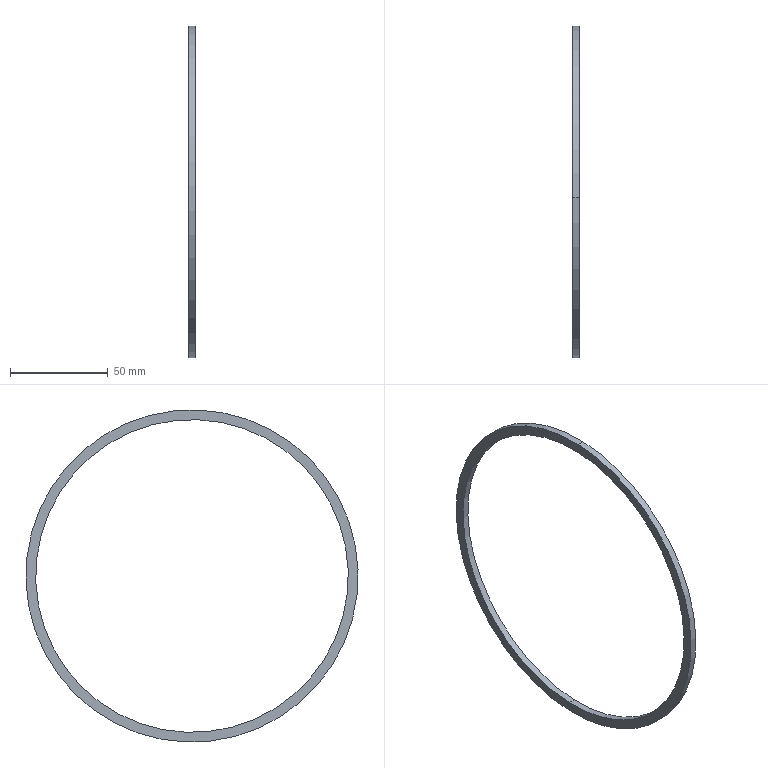Component | SolidWorks | SealRing2-1 | 1 solid | 6 faces | box 3.5 x 170 x 170 mm | volume 9071 mm3 | cylinder 4 | plane 2 | commonest cylinder face diameters 160 x2 170 x2
build123d program:
from build123d import *

# Parameters (mm, degrees)
SKETCH2_R           = 85
SKETCH2_R_2         = 80
BOSS_EXTRUDE1_DEPTH = 3.5


with BuildPart() as part:
    # Sketch2 → Boss-Extrude1 (new body)
    with BuildSketch(Plane(origin=(0, 0, 0), x_dir=(0, 0, -1), z_dir=(1, 0, 0))):
        Circle(SKETCH2_R)
        Circle(SKETCH2_R_2, mode=Mode.SUBTRACT)
    extrude(amount=BOSS_EXTRUDE1_DEPTH)


solid = part.part

# Placed as in the assembly
solid = solid.moved(Location((-63.5, 0, 0), (0, 0, 0)))
STEP:
#1=CARTESIAN_POINT('',(-2.362,-0.1192,3.147));
#2=VERTEX_POINT('',#1);
#3=CARTESIAN_POINT('',(-2.362,0.1192,-3.147));
#4=VERTEX_POINT('',#3);
#5=CARTESIAN_POINT('',(-2.362,-0.,-0.));
#6=DIRECTION('',(1.,0.,0.));
#7=DIRECTION('',(0.,0.03784,-0.9993));
#8=AXIS2_PLACEMENT_3D('',#5,#6,#7);
#9=CIRCLE('',#8,3.15);
#10=EDGE_CURVE('',#2,#4,#9,.T.);
#11=ORIENTED_EDGE('',*,*,#10,.T.);
#12=CARTESIAN_POINT('',(-2.5,0.1192,-3.147));
#13=VERTEX_POINT('',#12);
#14=CARTESIAN_POINT('',(-2.362,0.1192,-3.147));
#15=DIRECTION('',(-1.,0.,0.));
#16=VECTOR('',#15,39.37);
#17=LINE('',#14,#16);
#18=EDGE_CURVE('',#4,#13,#17,.T.);
#19=ORIENTED_EDGE('',*,*,#18,.T.);
#20=CARTESIAN_POINT('',(-2.5,-0.1192,3.147));
#21=VERTEX_POINT('',#20);
#22=CARTESIAN_POINT('',(-2.5,-0.,-0.));
#23=DIRECTION('',(1.,0.,0.));
#24=DIRECTION('',(0.,0.03784,-0.9993));
#25=AXIS2_PLACEMENT_3D('',#22,#23,#24);
#26=CIRCLE('',#25,3.15);
#27=EDGE_CURVE('',#21,#13,#26,.T.);
#28=ORIENTED_EDGE('',*,*,#27,.F.);
#29=CARTESIAN_POINT('',(-2.362,-0.1192,3.147));
#30=DIRECTION('',(-1.,0.,0.));
#31=VECTOR('',#30,39.37);
#32=LINE('',#29,#31);
#33=EDGE_CURVE('',#2,#21,#32,.T.);
#34=ORIENTED_EDGE('',*,*,#33,.F.);
#35=EDGE_LOOP('',(#11,#19,#28,#34));
#36=FACE_OUTER_BOUND('',#35,.T.);
#37=CARTESIAN_POINT('',(-2.362,-0.,-0.));
#38=DIRECTION('',(-1.,0.,0.));
#39=DIRECTION('',(0.,-0.03784,0.9993));
#40=AXIS2_PLACEMENT_3D('',#37,#38,#39);
#41=CYLINDRICAL_SURFACE('',#40,3.15);
#42=ADVANCED_FACE('',(#36),#41,.F.);
#43=CARTESIAN_POINT('',(-2.362,0.1266,-3.344));
#44=VERTEX_POINT('',#43);
#45=CARTESIAN_POINT('',(-2.362,-0.1266,3.344));
#46=VERTEX_POINT('',#45);
#47=CARTESIAN_POINT('',(-2.362,-0.,-0.));
#48=DIRECTION('',(1.,0.,0.));
#49=DIRECTION('',(0.,0.03784,-0.9993));
#50=AXIS2_PLACEMENT_3D('',#47,#48,#49);
#51=CIRCLE('',#50,3.346);
#52=EDGE_CURVE('',#44,#46,#51,.T.);
#53=ORIENTED_EDGE('',*,*,#52,.F.);
#54=CARTESIAN_POINT('',(-2.5,0.1266,-3.344));
#55=VERTEX_POINT('',#54);
#56=CARTESIAN_POINT('',(-2.362,0.1266,-3.344));
#57=DIRECTION('',(-1.,0.,0.));
#58=VECTOR('',#57,39.37);
#59=LINE('',#56,#58);
#60=EDGE_CURVE('',#44,#55,#59,.T.);
#61=ORIENTED_EDGE('',*,*,#60,.T.);
#62=CARTESIAN_POINT('',(-2.5,-0.1266,3.344));
#63=VERTEX_POINT('',#62);
#64=CARTESIAN_POINT('',(-2.5,-0.,-0.));
#65=DIRECTION('',(1.,0.,0.));
#66=DIRECTION('',(0.,0.03784,-0.9993));
#67=AXIS2_PLACEMENT_3D('',#64,#65,#66);
#68=CIRCLE('',#67,3.346);
#69=EDGE_CURVE('',#55,#63,#68,.T.);
#70=ORIENTED_EDGE('',*,*,#69,.T.);
#71=CARTESIAN_POINT('',(-2.362,-0.1266,3.344));
#72=DIRECTION('',(-1.,0.,0.));
#73=VECTOR('',#72,39.37);
#74=LINE('',#71,#73);
#75=EDGE_CURVE('',#46,#63,#74,.T.);
#76=ORIENTED_EDGE('',*,*,#75,.F.);
#77=EDGE_LOOP('',(#53,#61,#70,#76));
#78=FACE_OUTER_BOUND('',#77,.T.);
#79=CARTESIAN_POINT('',(-2.362,-0.,-0.));
#80=DIRECTION('',(-1.,0.,0.));
#81=DIRECTION('',(0.,-0.03784,0.9993));
#82=AXIS2_PLACEMENT_3D('',#79,#80,#81);
#83=CYLINDRICAL_SURFACE('',#82,3.346);
#84=ADVANCED_FACE('',(#78),#83,.T.);
#85=CARTESIAN_POINT('',(-2.362,-0.,-0.));
#86=DIRECTION('',(1.,0.,0.));
#87=DIRECTION('',(0.,0.03784,-0.9993));
#88=AXIS2_PLACEMENT_3D('',#85,#86,#87);
#89=CIRCLE('',#88,3.346);
#90=EDGE_CURVE('',#46,#44,#89,.T.);
#91=ORIENTED_EDGE('',*,*,#90,.T.);
#92=ORIENTED_EDGE('',*,*,#52,.T.);
#93=EDGE_LOOP('',(#91,#92));
#94=FACE_OUTER_BOUND('',#93,.T.);
#95=ORIENTED_EDGE('',*,*,#10,.F.);
#96=CARTESIAN_POINT('',(-2.362,-0.,-0.));
#97=DIRECTION('',(1.,0.,0.));
#98=DIRECTION('',(0.,0.03784,-0.9993));
#99=AXIS2_PLACEMENT_3D('',#96,#97,#98);
#100=CIRCLE('',#99,3.15);
#101=EDGE_CURVE('',#4,#2,#100,.T.);
#102=ORIENTED_EDGE('',*,*,#101,.F.);
#103=EDGE_LOOP('',(#95,#102));
#104=FACE_BOUND('',#103,.T.);
#105=CARTESIAN_POINT('',(-2.362,-0.,-0.));
#106=DIRECTION('',(1.,0.,0.));
#107=DIRECTION('',(0.,0.03784,-0.9993));
#108=AXIS2_PLACEMENT_3D('',#105,#106,#107);
#109=PLANE('',#108);
#110=ADVANCED_FACE('',(#94,#104),#109,.T.);
#111=CARTESIAN_POINT('',(-2.5,-0.,-0.));
#112=DIRECTION('',(1.,0.,0.));
#113=DIRECTION('',(0.,0.03784,-0.9993));
#114=AXIS2_PLACEMENT_3D('',#111,#112,#113);
#115=CIRCLE('',#114,3.346);
#116=EDGE_CURVE('',#63,#55,#115,.T.);
#117=ORIENTED_EDGE('',*,*,#116,.F.);
#118=ORIENTED_EDGE('',*,*,#69,.F.);
#119=EDGE_LOOP('',(#117,#118));
#120=FACE_OUTER_BOUND('',#119,.T.);
#121=ORIENTED_EDGE('',*,*,#27,.T.);
#122=CARTESIAN_POINT('',(-2.5,-0.,-0.));
#123=DIRECTION('',(1.,0.,0.));
#124=DIRECTION('',(0.,0.03784,-0.9993));
#125=AXIS2_PLACEMENT_3D('',#122,#123,#124);
#126=CIRCLE('',#125,3.15);
#127=EDGE_CURVE('',#13,#21,#126,.T.);
#128=ORIENTED_EDGE('',*,*,#127,.T.);
#129=EDGE_LOOP('',(#121,#128));
#130=FACE_BOUND('',#129,.T.);
#131=CARTESIAN_POINT('',(-2.5,-0.,-0.));
#132=DIRECTION('',(1.,0.,0.));
#133=DIRECTION('',(0.,0.03784,-0.9993));
#134=AXIS2_PLACEMENT_3D('',#131,#132,#133);
#135=PLANE('',#134);
#136=ADVANCED_FACE('',(#120,#130),#135,.F.);
#137=ORIENTED_EDGE('',*,*,#60,.F.);
#138=ORIENTED_EDGE('',*,*,#90,.F.);
#139=ORIENTED_EDGE('',*,*,#75,.T.);
#140=ORIENTED_EDGE('',*,*,#116,.T.);
#141=EDGE_LOOP('',(#137,#138,#139,#140));
#142=FACE_OUTER_BOUND('',#141,.T.);
#143=CARTESIAN_POINT('',(-2.362,-0.,-0.));
#144=DIRECTION('',(-1.,0.,0.));
#145=DIRECTION('',(0.,-0.03784,0.9993));
#146=AXIS2_PLACEMENT_3D('',#143,#144,#145);
#147=CYLINDRICAL_SURFACE('',#146,3.346);
#148=ADVANCED_FACE('',(#142),#147,.T.);
#149=ORIENTED_EDGE('',*,*,#18,.F.);
#150=ORIENTED_EDGE('',*,*,#101,.T.);
#151=ORIENTED_EDGE('',*,*,#33,.T.);
#152=ORIENTED_EDGE('',*,*,#127,.F.);
#153=EDGE_LOOP('',(#149,#150,#151,#152));
#154=FACE_OUTER_BOUND('',#153,.T.);
#155=CARTESIAN_POINT('',(-2.362,-0.,-0.));
#156=DIRECTION('',(-1.,0.,0.));
#157=DIRECTION('',(0.,-0.03784,0.9993));
#158=AXIS2_PLACEMENT_3D('',#155,#156,#157);
#159=CYLINDRICAL_SURFACE('',#158,3.15);
#160=ADVANCED_FACE('',(#154),#159,.F.);
#161=CLOSED_SHELL('',(#42,#84,#110,#136,#148,#160));
#162=MANIFOLD_SOLID_BREP('',#161);
#163=CARTESIAN_POINT('',(0.,0.,0.));
#164=DIRECTION('',(0.,0.,1.));
#165=DIRECTION('',(1.,0.,0.));
#166=AXIS2_PLACEMENT_3D('',#163,#164,#165);
#167=(LENGTH_UNIT()NAMED_UNIT(*)SI_UNIT($,.METRE.));
#168=LENGTH_MEASURE_WITH_UNIT(LENGTH_MEASURE(0.0254),#167);
#169=DIMENSIONAL_EXPONENTS(1.,0.,0.,0.,0.,0.,0.);
#170=(CONVERSION_BASED_UNIT('',#168)LENGTH_UNIT()NAMED_UNIT(#169));
#171=UNCERTAINTY_MEASURE_WITH_UNIT(LENGTH_MEASURE(0.00001),#170,'','');
#172=(NAMED_UNIT(*)PLANE_ANGLE_UNIT()SI_UNIT($,.RADIAN.));
#173=(NAMED_UNIT(*)SI_UNIT($,.STERADIAN.)SOLID_ANGLE_UNIT());
#174=(GEOMETRIC_REPRESENTATION_CONTEXT(3)GLOBAL_UNCERTAINTY_ASSIGNED_CONTEXT((#171))GLOBAL_UNIT_ASSIGNED_CONTEXT((#170,#172,#173))REPRESENTATION_CONTEXT('',''));
#175=ADVANCED_BREP_SHAPE_REPRESENTATION('',(#162,#166),#174);
#176=COLOUR_RGB('',0.7922,0.8196,0.9333);
#177=FILL_AREA_STYLE_COLOUR('',#176);
#178=FILL_AREA_STYLE('',(#177));
#179=SURFACE_STYLE_FILL_AREA(#178);
#180=SURFACE_SIDE_STYLE('',(#179));
#181=SURFACE_STYLE_USAGE(.BOTH.,#180);
#182=PRESENTATION_STYLE_ASSIGNMENT((#181));
#183=STYLED_ITEM('',(#182),#162);
#184=(LENGTH_UNIT()NAMED_UNIT(*)SI_UNIT($,.METRE.));
#185=LENGTH_MEASURE_WITH_UNIT(LENGTH_MEASURE(0.0254),#184);
#186=DIMENSIONAL_EXPONENTS(1.,0.,0.,0.,0.,0.,0.);
#187=(CONVERSION_BASED_UNIT('',#185)LENGTH_UNIT()NAMED_UNIT(#186));
#188=UNCERTAINTY_MEASURE_WITH_UNIT(LENGTH_MEASURE(0.00001),#187,'','');
#189=(NAMED_UNIT(*)PLANE_ANGLE_UNIT()SI_UNIT($,.RADIAN.));
#190=(NAMED_UNIT(*)SI_UNIT($,.STERADIAN.)SOLID_ANGLE_UNIT());
#191=(GEOMETRIC_REPRESENTATION_CONTEXT(3)GLOBAL_UNCERTAINTY_ASSIGNED_CONTEXT((#188))GLOBAL_UNIT_ASSIGNED_CONTEXT((#187,#189,#190))REPRESENTATION_CONTEXT('',''));
#192=MECHANICAL_DESIGN_GEOMETRIC_PRESENTATION_REPRESENTATION('',(#183),#191);
#193=PRESENTATION_LAYER_ASSIGNMENT('','',(#183));